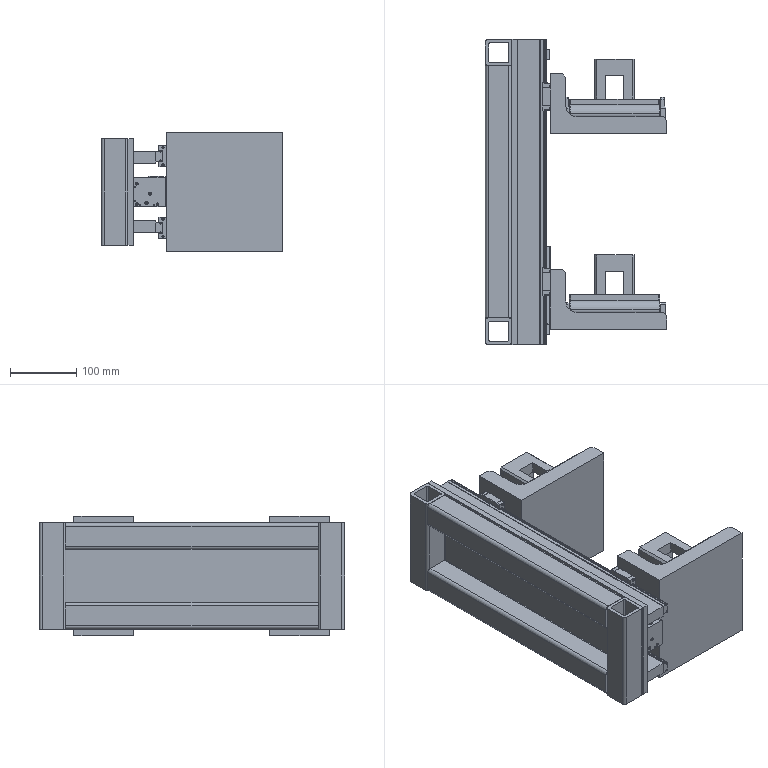Assembly | SolidWorks | mm | 45 component files | 45 solids | 2352 faces | box 273 x 460 x 180 mm | volume 4870522 mm3 | plane 1408 | cylinder 746 | cone 190 | torus 8 | commonest cylinder face diameters 3.5 x104 10 x56 6 x49 11 x48 3 x40 5 x36 4 x32 2.459 x32
Bill of materials:
40-40SquareTube7 | 2 |  | Long, straight hollow tube with a square cross-section and open ends.
40-40SquareTube8 | 2 |  | Short hollow tube with a square cross-section and open ends. Its profile looks the same as the long square tube, but it is cut shorter relative to its width.
532446 DGC-182804---00041181--(ZR) | 1 |  | Long, straight extruded bar with a complex, uneven cross-section. It has a large off-centre round bore and several undercut slots and notches around its edges.
532446 DGC-18-G-PG---(SG)_1 | 1 |  | Extruded profile segment. The end profile shows an upper cap with a rounded top surface over a lower body containing a C-shaped channel. One side face has two small circular holes.
HI_532446 DGC-18-G---(0DL)_1 | 1 |  | Rectangular block with rounded edges. It has a central through-hole on its large face, holes on its top face, and an angled shallow recess near one edge.
HI_532446 DGC-18-G---(0DR)_1 | 1 |  | Rectangular block with rounded edges and many holes. Several blind holes with drill-point bottoms sit near the corners, and there are additional through-holes and holes on the top face.
HI_DIN-913 - M5x5_1 | 4 |  | Short solid cylinder with a hexagonal socket in one end. Both ends are chamfered, and the opposite end has a pronounced conical chamfer.
DualStationFixturePlate | 2 |  | Thin, flat, nearly square plate with small corner chamfers. It has one large central hole and two smaller holes at opposite diagonal corners.
LocatingBlock | 4 |  | Cube-like open-frame bracket. One face is a square with chamfered corners and a hole near each corner; behind it, four projecting square arms end in drilled holes. It also has a central round opening, a large U-shaped cutout, and a rounded rectangular slot.
Set | 4 |  | Short cylindrical sleeve or ring with a fairly thin wall and a smooth bore. The edges at one or both ends are chamfered.
L-Plate | 2 |  | Short L-shaped angle section. It has a large fillet in the inside corner, chamfered leg tips, and small step features near the ends of one leg.
Roller | 6 |  | Stepped solid shaft: a long main cylinder with a smaller coaxial pin at each end. The shoulder edges have small chamfers.
RollerMountingPlate | 4 |  | Flat rectangular bar/plate with three evenly spaced round through-holes in a single row, offset toward one long edge; small corner chamfers on that same long edge at both ends.
r_SEBV16-630 | 2 |  | Long, slender straight bar of constant cross-section with a necked profile (a slot-like recess on each side under a wider top) and a single row of evenly spaced round holes along its length.
SEBV16_b | 4 |  | Rectangular block body with a stepped channel through its underside, thinner end plates on both ends, four round holes in a rectangular pattern on the main face, and two straight longitudinal grooves between the hole rows.
SlideRailShim | 2 |  | Plain solid rectangular bar (square-ended prism) with no holes, chamfers or other visible features.
StopPlate2 | 2 |  | Elongated rectangular bar of near-square or rectangular section with chamfers on two corners at one end; no holes visible.
VerticalPlate | 1 |  | Thin flat rectangular plate/sheet with no holes, cutouts or edge features visible.
Mates:
1. coincident | 40-40SquareTube8-1 face at (1.398, 47.837, 180) dir (0, 1, 0) | 40-40SquareTube7-1 face at (32.398, 47.837, 145) dir (0, -1, 0)
2. coincident | 40-40SquareTube8-1 edge at (37.398, 11.837, 180) dir (0, 1, 0) | 40-40SquareTube7-1 face at (32.398, 427.837, 180) dir (0, 0, 1)
3. coincident | 40-40SquareTube8-1 face at (37.398, 11.837, 180) dir (1, 0, 0) | 40-40SquareTube7-1 face at (37.398, 427.837, 175) dir (1, 0, 0)
4. coincident | 40-40SquareTube8-1 face at (1.398, 47.837, 180) dir (0, 1, 0) | 40-40SquareTube7-2 face at (32.398, 47.837, 25) dir (0, -1, 0)
5. coincident | 40-40SquareTube8-1 face at (37.398, 11.837, 180) dir (1, 0, 0) | 40-40SquareTube7-2 face at (37.398, 427.837, 55) dir (1, 0, 0)
6. coincident | 40-40SquareTube8-1 face at (33.398, 11.837, 20) dir (0, 0, -1) | 40-40SquareTube7-2 face at (32.398, 427.837, 20) dir (0, 0, -1)
7. coincident | 40-40SquareTube7-1 face at (32.398, 427.837, 145) dir (0, 1, 0) | 40-40SquareTube8-2 face at (1.398, 427.837, 180) dir (0, -1, 0)
8. coincident | 40-40SquareTube7-1 face at (37.398, 427.837, 175) dir (1, 0, 0) | 40-40SquareTube8-2 face at (37.398, 431.837, 180) dir (1, 0, 0)
9. coincident | 40-40SquareTube7-1 face at (32.398, 427.837, 180) dir (0, 0, 1) | 40-40SquareTube8-2 face at (33.398, 431.837, 180) dir (0, 0, 1)
10. coincident | 40-40SquareTube8-1 face at (37.398, 11.837, 180) dir (1, 0, 0) | VerticalPlate-1 face at (37.398, 237.837, 100) dir (-1, 0, 0)
11. distance | 40-40SquareTube8-1 face at (1.398, 47.837, 180) dir (0, 1, 0) | VerticalPlate-1 face at (37.398, 7.837, 180) dir (0, -1, 0)
12. coincident | 40-40SquareTube8-2 plane at (17.398, 447.837, 100) dir (0, 0, 1) | VerticalPlate-1 plane at (41.398, 237.837, 100) dir (0, 0, 1)
13. coincident | VerticalPlate-1 plane at (41.398, 237.837, 100) dir (0, 0, 1) | L-Plate-1 plane at (95.398, 325.813, 100) dir (0, 0, -1)
14. distance | SEBV16-630_2_03-1/SEBV16_b-1 face at (94.898, 367.437, 170) dir (0, 0, 1) | VerticalPlate-1 face at (37.398, 7.837, 180) dir (0, 0, 1)
15. distance | SEBV16-630_2_03-2/SEBV16_b-1 face at (83.898, 367.437, 30) dir (0, 0, -1) | VerticalPlate-1 face at (37.398, 7.837, 20) dir (0, 0, -1)
16. coincident | SEBV16-630_2_03-1/SEBV16_b-1 face at (95.398, 367.437, 161.8) dir (1, 0, 0) | L-Plate-1 face at (95.398, 415.813, 10) dir (-1, 0, 0)
17. distance | VerticalPlate-1 face at (45.398, 237.837, 100) dir (1, 0, 0) | SEBV16-630_2_03-1/r_SEBV16-630-1 face at (79.398, 7.837, 161) dir (-1, 0, 0)
18. distance | VerticalPlate-1 face at (45.398, 237.837, 100) dir (1, 0, 0) | SEBV16-630_2_03-2/r_SEBV16-630-1 face at (79.398, 7.837, 53) dir (-1, 0, 0)
19. coincident | VerticalPlate-1 face at (37.398, 7.837, 180) dir (0, -1, 0) | SEBV16-630_2_03-1/r_SEBV16-630-1 face at (86.513, 7.837, 146.185) dir (0, -1, 0)
20. coincident | VerticalPlate-1 face at (37.398, 7.837, 180) dir (0, -1, 0) | SEBV16-630_2_03-2/r_SEBV16-630-1 face at (86.513, 7.837, 38.185) dir (0, -1, 0)
21. coincident | L-Plate-1 face at (270.398, 335.813, 10) dir (0, 1, 0) | RollerMountingPlate-1 face at (115.398, 335.813, 30) dir (0, -1, 0)
22. distance | RollerMountingPlate-1 face at (115.398, 350.813, 100) dir (-1, 0, 0) | L-Plate-1 face at (105.398, 335.813, 10) dir (1, 0, 0)
23. coincident | L-Plate-1 plane at (95.398, 325.813, 100) dir (0, 0, -1) | RollerMountingPlate-1 plane at (119.398, 350.813, 100) dir (0, 0, -1)
24. concentric | RollerMountingPlate-1 face at (115.398, 355.813, 160) dir (1, 0, 0) r 5 | Roller-1 face at (269.398, 355.813, 160) dir (1, 0, 0) r 5
25. concentric | RollerMountingPlate-1 face at (115.398, 355.813, 100) dir (1, 0, 0) r 5 | Roller-7 face at (269.398, 355.813, 100) dir (1, 0, 0) r 5
26. coincident | Roller-1 face at (260.398, 356.284, 173.992) dir (1, 0, 0) | Roller-7 face at (260.398, 352.742, 113.659) dir (1, 0, 0)
27. concentric | RollerMountingPlate-1 face at (115.398, 355.813, 40) dir (1, 0, 0) r 5 | Roller-9 face at (269.398, 355.813, 40) dir (1, 0, 0) r 5
28. coincident | Roller-7 face at (260.398, 352.742, 113.659) dir (1, 0, 0) | Roller-9 face at (260.398, 359.651, 53.464) dir (1, 0, 0)
29. coincident | RollerMountingPlate-1 face at (115.398, 350.813, 100) dir (-1, 0, 0) | Roller-1 face at (115.398, 355.813, 160) dir (-1, 0, 0)
30. coincident | L-Plate-1 face at (270.398, 335.813, 10) dir (0, 1, 0) | RollerMountingPlate-5 face at (261.398, 335.813, 30) dir (0, -1, 0)
31. coincident | RollerMountingPlate-1 face at (115.398, 365.813, 170) dir (0, 0, 1) | RollerMountingPlate-5 face at (261.398, 365.813, 170) dir (0, 0, 1)
32. coincident | Roller-1 face at (269.398, 355.981, 164.997) dir (1, 0, 0) | RollerMountingPlate-5 face at (269.398, 350.813, 100) dir (1, 0, 0)
33. coincident | VerticalPlate-1 face at (45.398, 237.837, 100) dir (1, 0, 0) | SlideRailShim-2 face at (45.398, 237.837, 152.5) dir (-1, 0, 0)
34. coincident | SEBV16-630_2_03-1/r_SEBV16-630-1 face at (84.674, 7.837, 161.5) dir (0, 0, 1) | SlideRailShim-2 face at (45.398, 7.837, 161.5) dir (0, 0, 1)
35. coincident | SEBV16-630_2_03-1/r_SEBV16-630-1 face at (79.398, 467.837, 161.5) dir (0, 1, 0) | SlideRailShim-2 face at (45.398, 467.837, 161.5) dir (0, 1, 0)
36. coincident | VerticalPlate-1 face at (45.398, 237.837, 100) dir (1, 0, 0) | SlideRailShim-3 face at (45.398, 237.837, 47.5) dir (-1, 0, 0)
37. coincident | SEBV16-630_2_03-2/r_SEBV16-630-1 edge at (79.898, 7.837, 38.5) dir (0, 1, 0) | SlideRailShim-3 face at (45.398, 7.837, 38.5) dir (0, 0, -1)
38. coincident | SEBV16-630_2_03-2/r_SEBV16-630-1 face at (79.398, 467.837, 53.5) dir (0, 1, 0) | SlideRailShim-3 face at (45.398, 467.837, 56.5) dir (0, 1, 0)
39. distance | 40-40SquareTube8-2 face at (1.398, 467.837, 180) dir (0, 1, 0) | DGC-18-280-G-PPV-A-1/HI_532446 DGC-18-G---(0DL)_1-1 face at (88.798, 452.837, 88.55) dir (0, 1, 0)
40. coincident | VerticalPlate-1 face at (45.398, 237.837, 100) dir (1, 0, 0) | DGC-18-280-G-PPV-A-1/HI_532446 DGC-18-G---(0DL)_1-1 face at (45.398, 437.837, 79.237) dir (-1, 0, 0)
41. coincident | RollerMountingPlate-5 face at (261.398, 365.813, 30) dir (0, 1, 0) | StopPlate2-1 face at (267.398, 365.813, 165) dir (0, -1, 0)
42. distance | RollerMountingPlate-5 face at (269.398, 350.813, 100) dir (1, 0, 0) | StopPlate2-1 face at (267.398, 376.402, 98.988) dir (1, 0, 0)
43. distance | StopPlate2-1 face at (267.398, 365.813, 165) dir (0, 0, 1) | RollerMountingPlate-5 face at (261.398, 365.813, 170) dir (0, 0, 1)
44. coincident | RollerMountingPlate-1 face at (115.398, 365.813, 30) dir (0, 1, 0) | StopPlate2-3 face at (116.398, 365.813, 35) dir (0, -1, 0)
45. parallel | RollerMountingPlate-1 face at (123.398, 350.813, 100) dir (1, 0, 0) | StopPlate2-3 face at (122.398, 376.402, 101.012) dir (1, 0, 0)
46. distance | StopPlate2-3 face at (122.398, 376.402, 101.012) dir (1, 0, 0) | RollerMountingPlate-1 face at (123.398, 350.813, 100) dir (1, 0, 0)
47. coincident | StopPlate2-1 face at (267.398, 365.813, 35) dir (0, 0, -1) | StopPlate2-3 face at (116.398, 365.813, 35) dir (0, 0, -1)
48. tangent | Roller-7 face at (269.398, 355.813, 100) dir (1, 0, 0) r 14 | DualStationFixture-1/DualStationFixturePlate-2 face at (191.898, 369.813, 99.048) dir (0, -1, 0)
49. tangent | Roller-9 face at (269.398, 355.813, 40) dir (1, 0, 0) r 14 | DualStationFixture-1/DualStationFixturePlate-2 face at (191.898, 369.813, 99.048) dir (0, -1, 0)
50. parallel | StopPlate2-1 face at (267.398, 376.402, 98.988) dir (1, 0, 0) | DualStationFixture-1/DualStationFixturePlate-2 face at (259.898, 377.813, 34.048) dir (1, 0, 0)
51. distance | StopPlate2-1 face at (261.398, 376.402, 98.988) dir (-1, 0, 0) | DualStationFixture-1/DualStationFixturePlate-2 face at (259.898, 377.813, 34.048) dir (1, 0, 0)
52. tangent | Roller-8 face at (269.398, 60.813, 100) dir (1, 0, 0) r 14 | DualStationFixture-2/DualStationFixturePlate-2 face at (191.898, 74.813, 99.048) dir (0, -1, 0)
53. tangent | Roller-10 face at (269.398, 60.813, 40) dir (1, 0, 0) r 14 | DualStationFixture-2/DualStationFixturePlate-2 face at (191.898, 74.813, 99.048) dir (0, -1, 0)
54. coincident | DualStationFixture-1/DualStationFixturePlate-2 face at (259.898, 377.813, 34.048) dir (0, 0, -1) | DualStationFixture-2/DualStationFixturePlate-2 face at (259.898, 82.813, 34.048) dir (0, 0, -1)
55. coincident | DualStationFixture-1/DualStationFixturePlate-2 face at (259.898, 377.813, 34.048) dir (1, 0, 0) | DualStationFixture-2/DualStationFixturePlate-2 face at (259.898, 82.813, 34.048) dir (1, 0, 0)
56. coincident | DualStationFixturePlate-2 face at (-129.29, -24.163, -86.459) dir (0.8131, -0.3726, 0.4472) | LocatingBlock-1 face at (-128.031, 0.002167, -68.613) dir (-0.8131, 0.3726, -0.4472)
57. concentric | DualStationFixturePlate-2 face at (-112.621, -27.516, -137.448) dir (0.8131, -0.3726, 0.4472) r 5.5 | Set-1 face at (-112.455, -27.592, -137.357) dir (-0.8131, 0.3726, -0.4472) r 5.5
58. coincident | DualStationFixturePlate-2 face at (-129.29, -24.163, -86.459) dir (0.8131, -0.3726, 0.4472) | Set-1 face at (-109.004, -34.905, -132.292) dir (0.8131, -0.3726, 0.4472)
59. concentric | DualStationFixturePlate-2 face at (-158.969, -14.847, -42.625) dir (0.8131, -0.3726, 0.4472) r 5.5 | Set-3 face at (-158.803, -14.922, -42.534) dir (-0.8131, 0.3726, -0.4472) r 5.5
60. coincident | DualStationFixturePlate-2 face at (-129.29, -24.163, -86.459) dir (0.8131, -0.3726, 0.4472) | Set-3 face at (-155.649, -21.106, -35.988) dir (0.8131, -0.3726, 0.4472)
61. coincident | DualStationFixturePlate-2 plane at (-132.542, -22.672, -88.247) dir (0.003164, 0.7711, 0.6367) | LocatingBlock-1 plane at (-86.269, -18.82, -93.142) dir (0.003164, 0.7711, 0.6367)
62. coincident | DualStationFixturePlate-2 face at (-129.29, -24.163, -86.459) dir (0.8131, -0.3726, 0.4472) | LocatingBlock-2 face at (-165.287, -33.042, -28.412) dir (-0.8131, 0.3726, -0.4472)
63. coincident | LocatingBlock-1 plane at (-86.269, -18.82, -93.142) dir (0.003164, 0.7711, 0.6367) | LocatingBlock-2 plane at (-123.525, -51.864, -52.942) dir (0.003164, 0.7711, 0.6367)
64. distance | LocatingBlock-1 plane at (-86.269, -18.82, -93.142) dir (0.5821, 0.5163, -0.6281) | LocatingBlock-2 plane at (-123.525, -51.864, -52.942) dir (0.5821, 0.5163, -0.6281)
65. distance | LocatingBlock-1 plane at (-86.269, -18.82, -93.142) dir (0.5821, 0.5163, -0.6281) | DualStationFixturePlate-2 plane at (-132.542, -22.672, -88.247) dir (0.5821, 0.5163, -0.6281)
66. distance | SEBV16_b-1 face at (-87.445, 17.539, -44.6) dir (0, 1, 0) | r_SEBV16-630-1 face at (-83.445, 11.039, 315) dir (0, 1, 0)
67. distance | SEBV16_b-1 face at (-74.645, 6.039, -44.6) dir (1, 0, 0) | r_SEBV16-630-1 face at (-83.145, 2.039, 315) dir (1, 0, 0)
68. distance | SEBV16_b-1 face at (-90.645, 1.539, -79) dir (0, 0, -1) | r_SEBV16-630-1 face at (-98.145, 1.539, -145) dir (0, 0, -1)
69. coincident | r_SEBV16-630-1 face at (-83.445, 11.039, 315) dir (0, 1, 0) | SEBV16_b-2 face at (-83.445, 11.039, 234.304) dir (0, -1, 0)
70. coincident | SEBV16_b-1 face at (-74.645, 6.039, -44.6) dir (1, 0, 0) | SEBV16_b-2 face at (-74.645, 6.039, 234.304) dir (1, 0, 0)